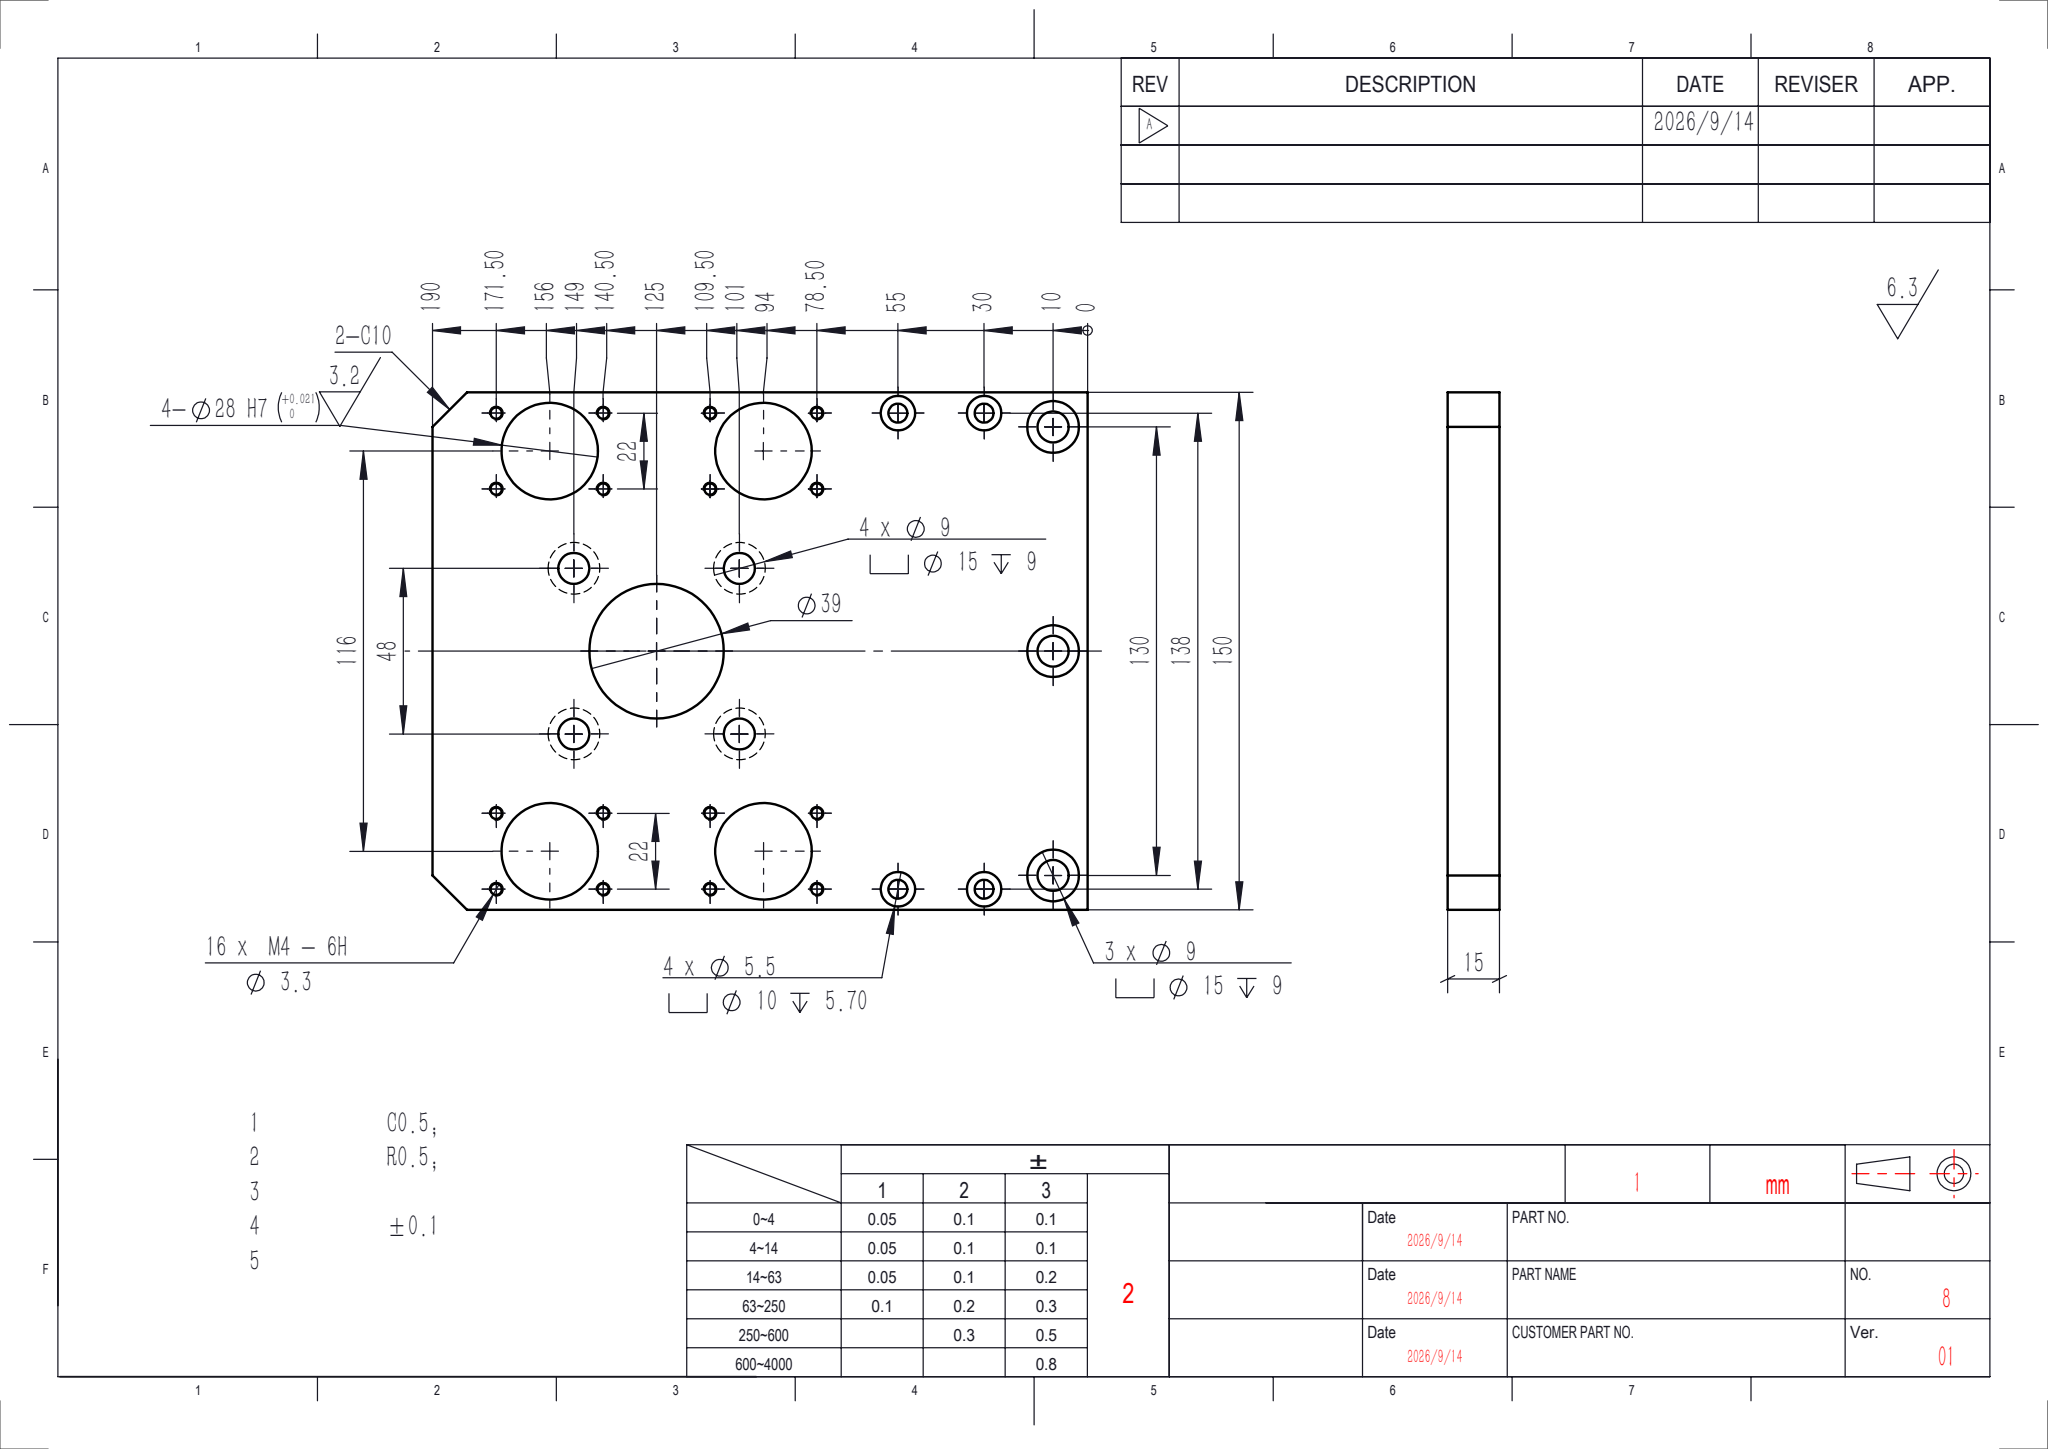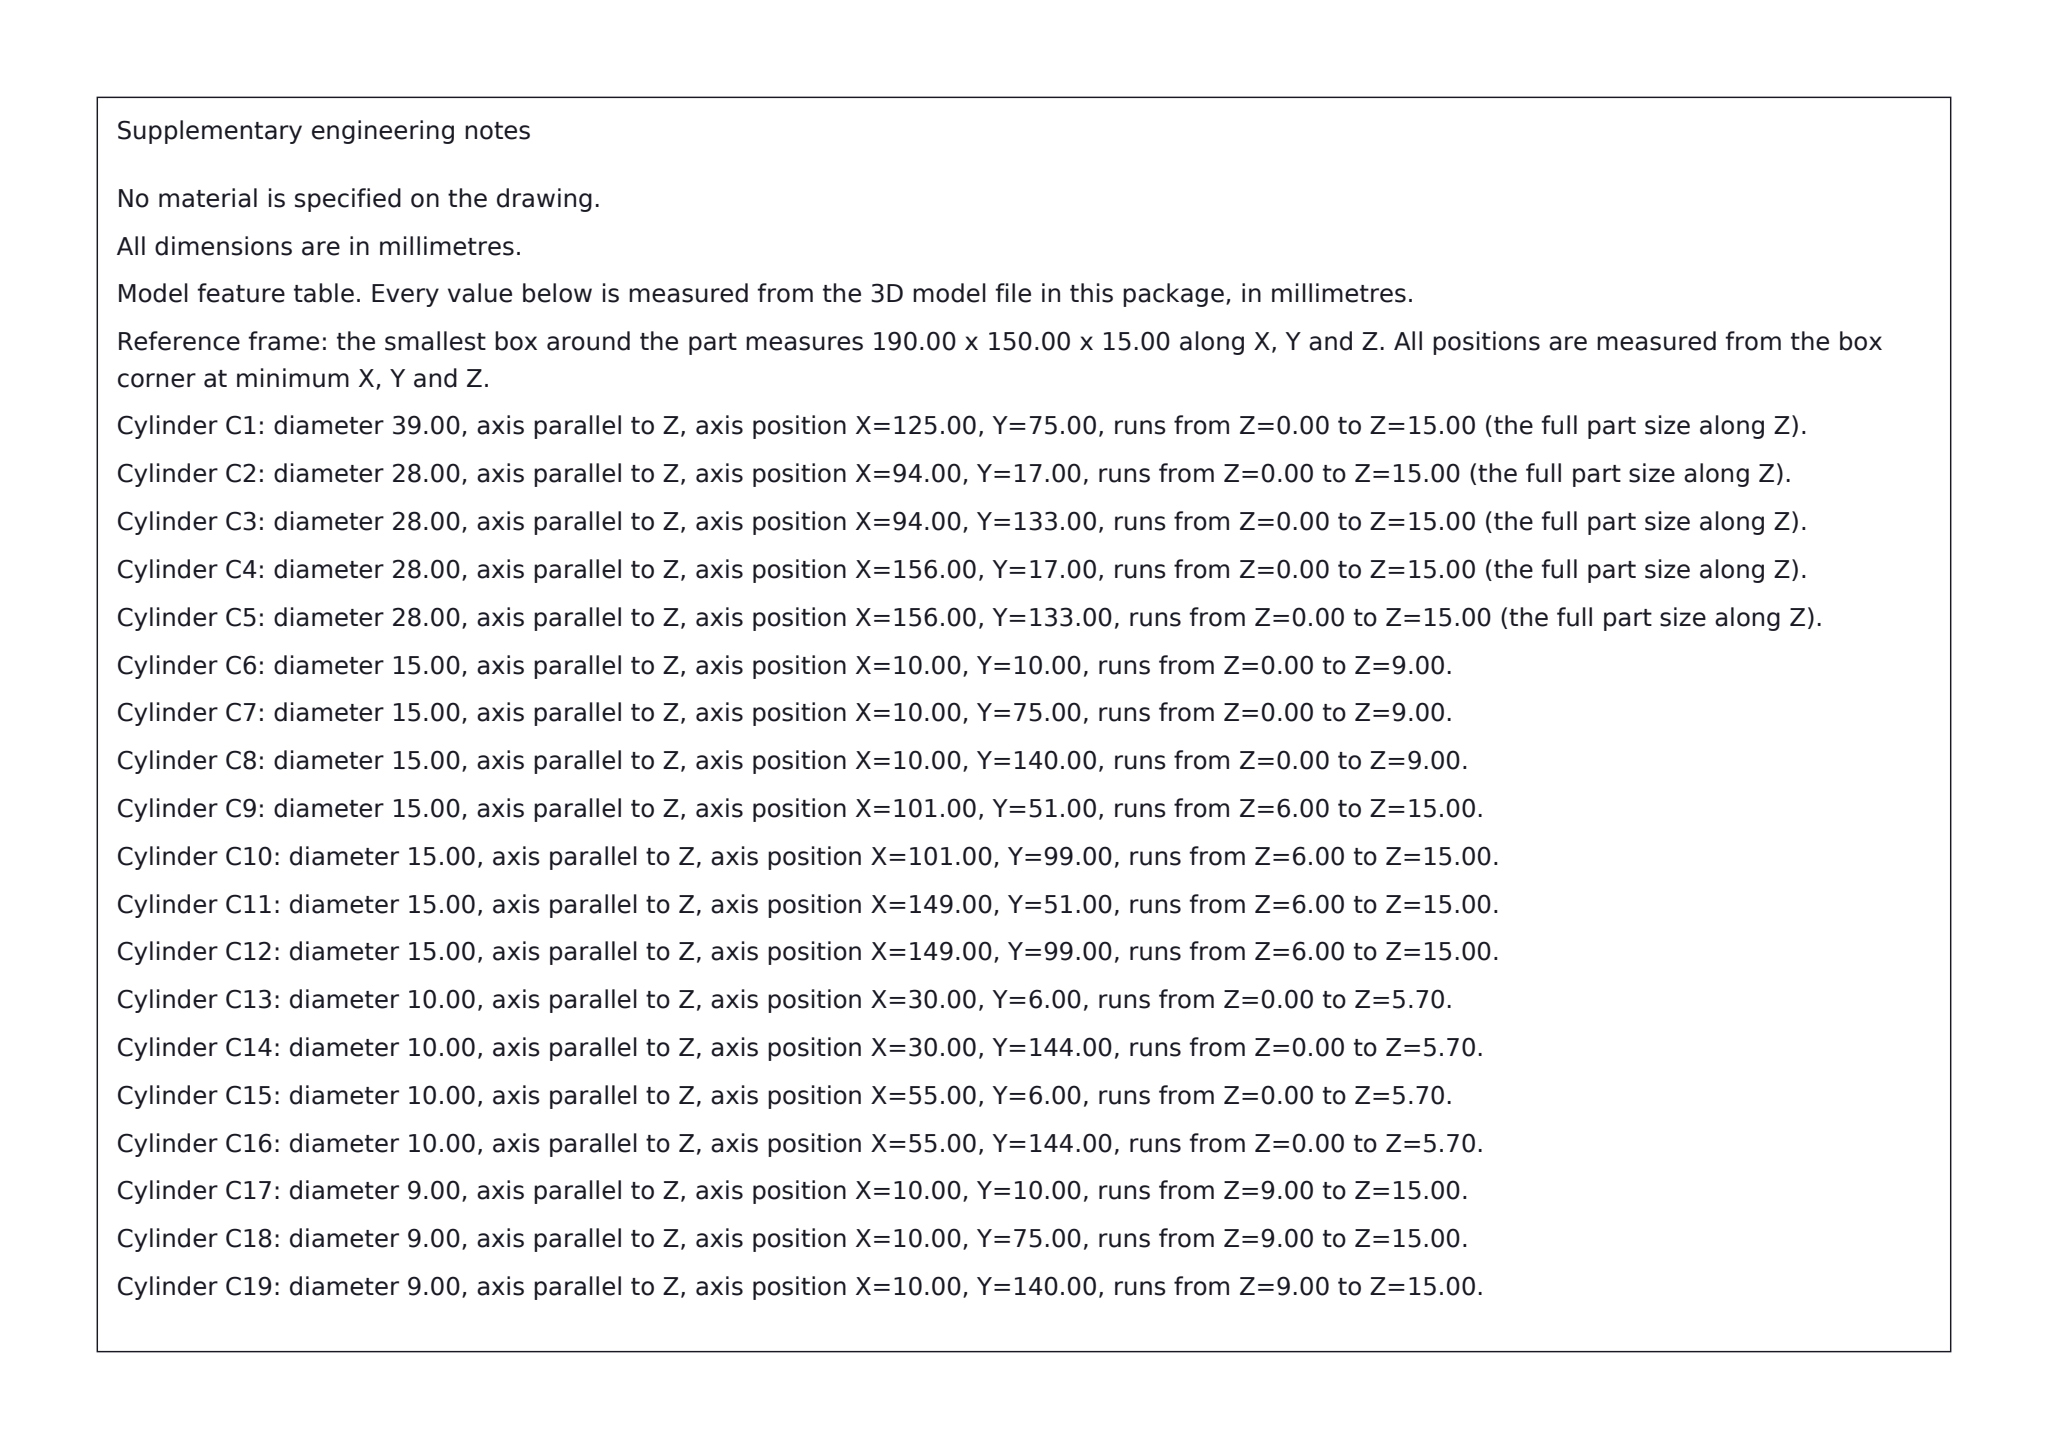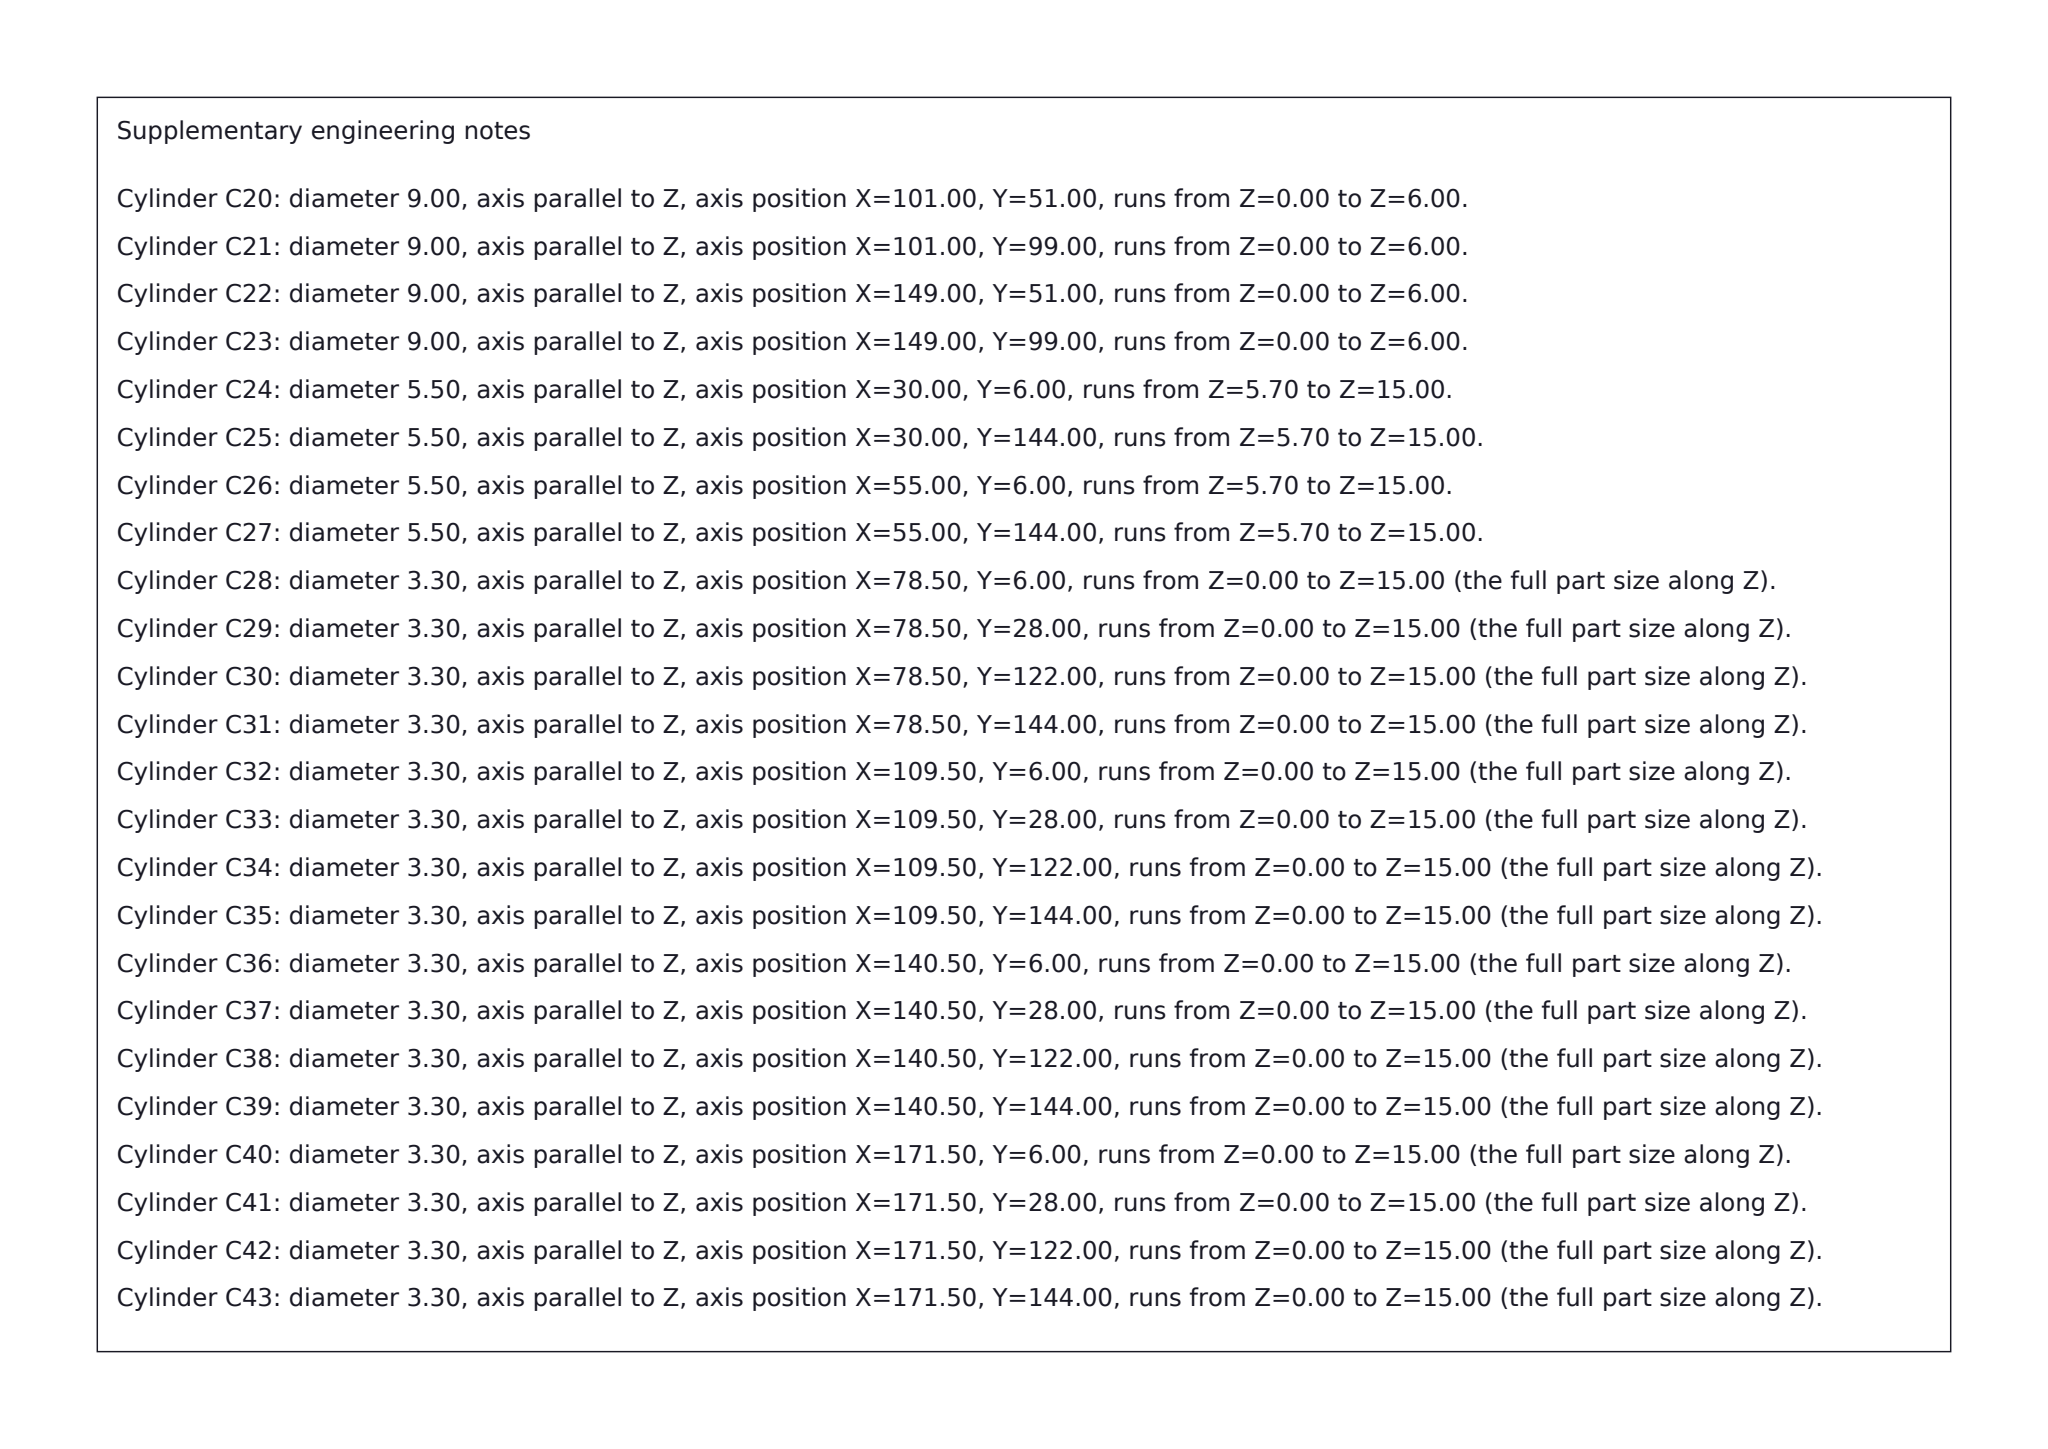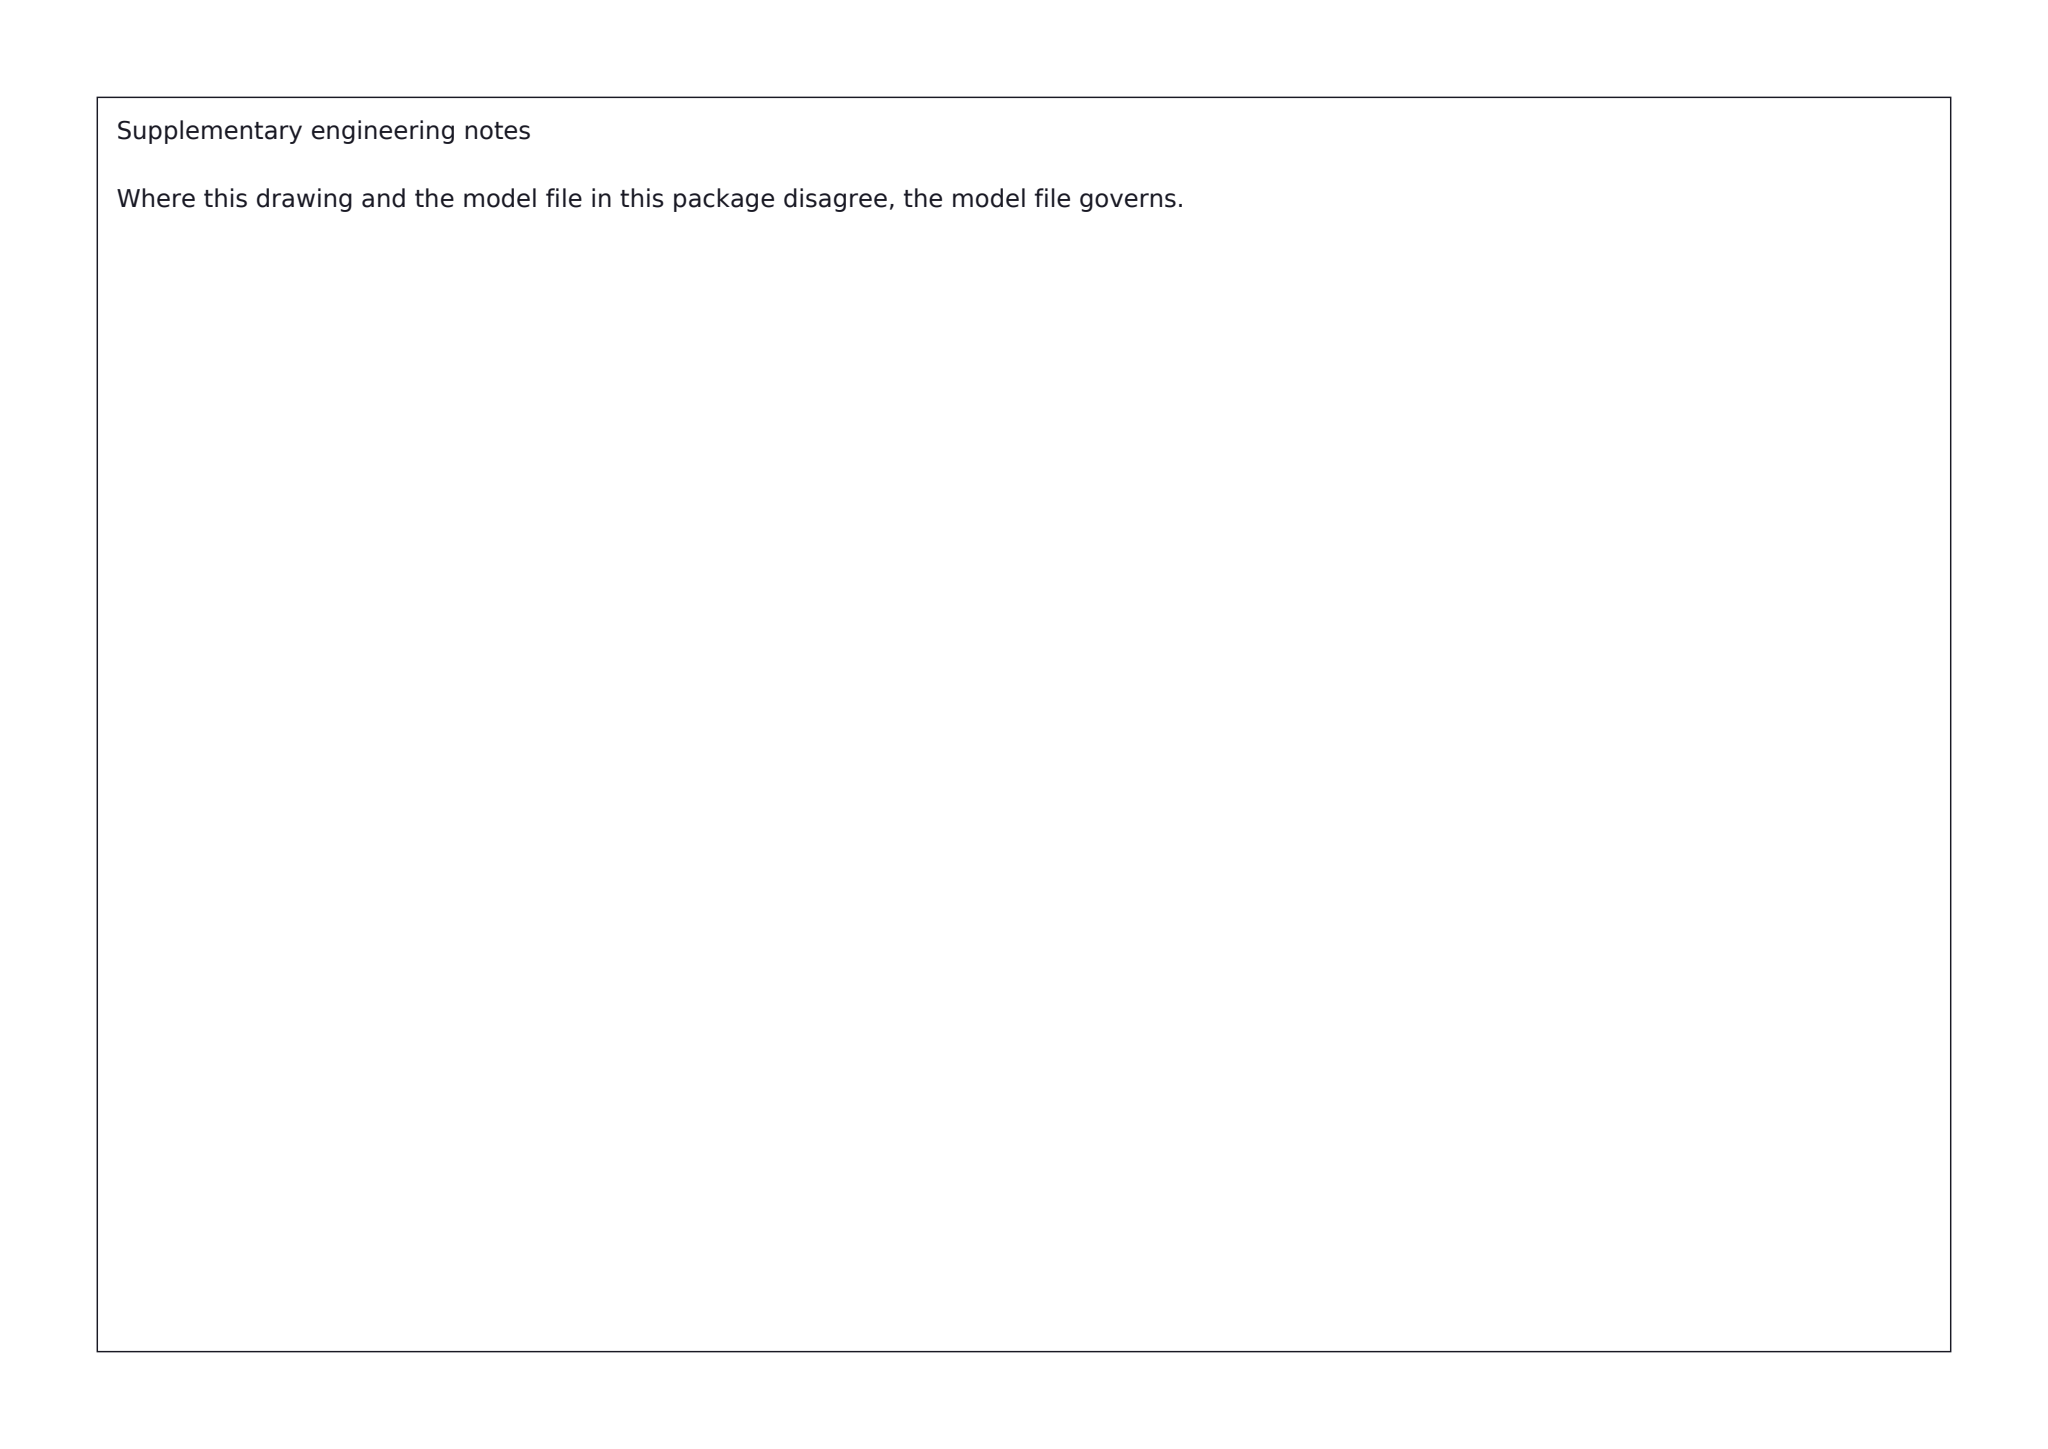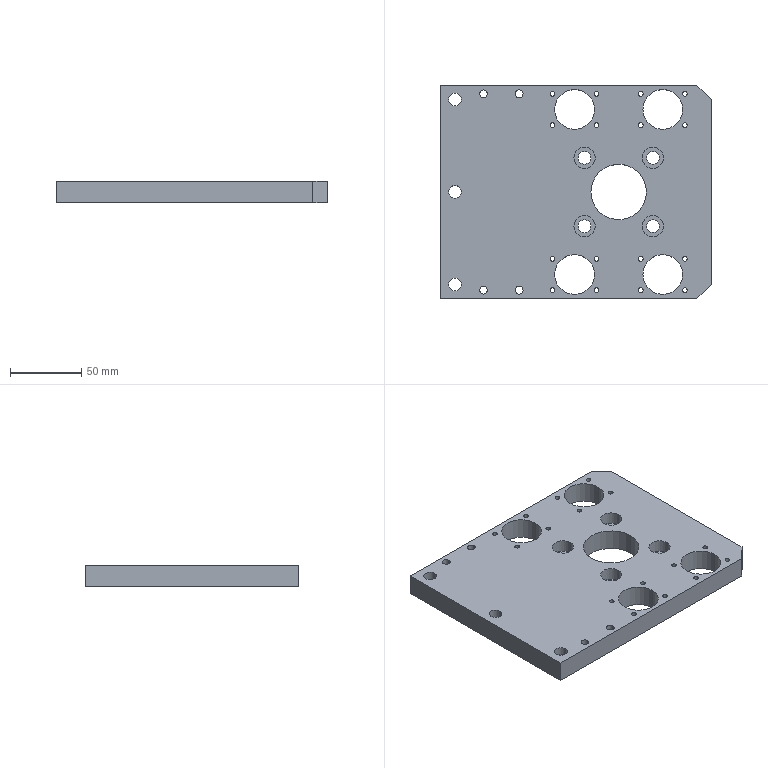Part | SolidWorks | mm | 1 solid | 105 faces | box 190 x 150 x 15 mm | volume 352604 mm3 | cylinder 86 | plane 19 | commonest cylinder face diameters 3.3 x32 15 x14 9 x14 10 x8 5.5 x8 28 x8 39 x2
build123d program:
from build123d import *

# Parameters (mm, degrees)
SKETCH1_W                                            = 190
SKETCH1_H                                            = 150
BOSS_EXTRUDE1_DEPTH                                  = 15
SKETCH2_R                                            = 19.5
CUT_EXTRUDE1_DEPTH                                   = 122.963
HOLE_SIZE_ACCORDING_TO_THE_TYPE_OF_HEXAG_D           = 9
HOLE_SIZE_ACCORDING_TO_THE_TYPE_OF_HEXAG_CBORE_D     = 15
HOLE_SIZE_ACCORDING_TO_THE_TYPE_OF_HEXAG_CBORE_DEPTH = 9
SKETCH6_R                                            = 14
CUT_EXTRUDE2_DEPTH                                   = 122.963
M4_TAPPED_HOLE1_D                                    = 3.3
LPATTERN1_COUNT                                      = 2
LPATTERN1_PITCH                                      = 62
LPATTERN1_COUNT_DIR2                                 = 2
LPATTERN1_PITCH_DIR2                                 = 116
HOLE_SIZE_ACCORDING_TO_THE_TYPE_OF_H_2_D             = 9
HOLE_SIZE_ACCORDING_TO_THE_TYPE_OF_H_2_CBORE_D       = 15
HOLE_SIZE_ACCORDING_TO_THE_TYPE_OF_H_2_CBORE_DEPTH   = 9
HOLE_SIZE_ACCORDING_TO_THE_TYPE_OF_H_3_D             = 5.5
HOLE_SIZE_ACCORDING_TO_THE_TYPE_OF_H_3_CBORE_D       = 10
HOLE_SIZE_ACCORDING_TO_THE_TYPE_OF_H_3_CBORE_DEPTH   = 5.7
CHAMFER1_SIZE                                        = 10


with BuildPart() as part:
    # Sketch1 → Boss-Extrude1 (new body)
    with BuildSketch(Plane.XY):
        Rectangle(SKETCH1_W, SKETCH1_H)
    extrude(amount=BOSS_EXTRUDE1_DEPTH)

    # Sketch2 → Cut-Extrude1 (cut, through all)
    with BuildSketch(Plane.XY.offset(15)):
        with Locations((30, 0)):
            Circle(SKETCH2_R)
    extrude(amount=-CUT_EXTRUDE1_DEPTH, mode=Mode.SUBTRACT)

    # Hole Size according to the type of Hexag (through all)
    with Locations(Plane.XY.offset(15)):
        with Locations((6, 24), (6, -24), (54, -24), (54, 24)):
            CounterBoreHole(HOLE_SIZE_ACCORDING_TO_THE_TYPE_OF_HEXAG_D / 2, HOLE_SIZE_ACCORDING_TO_THE_TYPE_OF_HEXAG_CBORE_D / 2, HOLE_SIZE_ACCORDING_TO_THE_TYPE_OF_HEXAG_CBORE_DEPTH)

    # Sketch6 → Cut-Extrude2 (cut, through all)
    with BuildSketch(Plane(origin=(0, 0, 0), x_dir=(-1, 0, 0), z_dir=(0, 0, -1))):
        with Locations((-61, 58)):
            Circle(SKETCH6_R)
    cut_extrude2 = extrude(amount=-CUT_EXTRUDE2_DEPTH, mode=Mode.SUBTRACT)

    # M4 Tapped Hole1 (through all)
    with Locations(Plane(origin=(0, 0, 0), x_dir=(-1, 0, 0), z_dir=(0, 0, -1))):
        with Locations((-76.5, 69), (-45.5, 69), (-45.5, 47), (-76.5, 47)):
            m4_tapped_hole1 = Hole(M4_TAPPED_HOLE1_D / 2)

    # LPattern1: Cut-Extrude2, M4 Tapped Hole1 2 × 2
    with Locations(*[(-i * LPATTERN1_PITCH, -j * LPATTERN1_PITCH_DIR2, 0) for i in range(LPATTERN1_COUNT) for j in range(LPATTERN1_COUNT_DIR2) if (i, j) != (0, 0)]):
        add(cut_extrude2, mode=Mode.SUBTRACT)
        add(m4_tapped_hole1, mode=Mode.SUBTRACT)

    # Hole Size according to the type of H 2 (through all)
    with Locations(Plane(origin=(0, 0, 0), x_dir=(-1, 0, 0), z_dir=(0, 0, -1))):
        with Locations((85, 65), (85, 0), (85, -65)):
            CounterBoreHole(HOLE_SIZE_ACCORDING_TO_THE_TYPE_OF_H_2_D / 2, HOLE_SIZE_ACCORDING_TO_THE_TYPE_OF_H_2_CBORE_D / 2, HOLE_SIZE_ACCORDING_TO_THE_TYPE_OF_H_2_CBORE_DEPTH)

    # Hole Size according to the type of H 3 (through all)
    with Locations(Plane(origin=(0, 0, 0), x_dir=(-1, 0, 0), z_dir=(0, 0, -1))):
        with Locations((40, 69), (65, 69), (65, -69), (40, -69)):
            CounterBoreHole(HOLE_SIZE_ACCORDING_TO_THE_TYPE_OF_H_3_D / 2, HOLE_SIZE_ACCORDING_TO_THE_TYPE_OF_H_3_CBORE_D / 2, HOLE_SIZE_ACCORDING_TO_THE_TYPE_OF_H_3_CBORE_DEPTH)

    # Chamfer1
    chamfer1_edges = [part.edges().sort_by_distance(p)[0] for p in [
        (95, -75, 7.5),
        (95, 75, 7.5),
    ]]
    chamfer(chamfer1_edges, length=CHAMFER1_SIZE)


solid = part.part